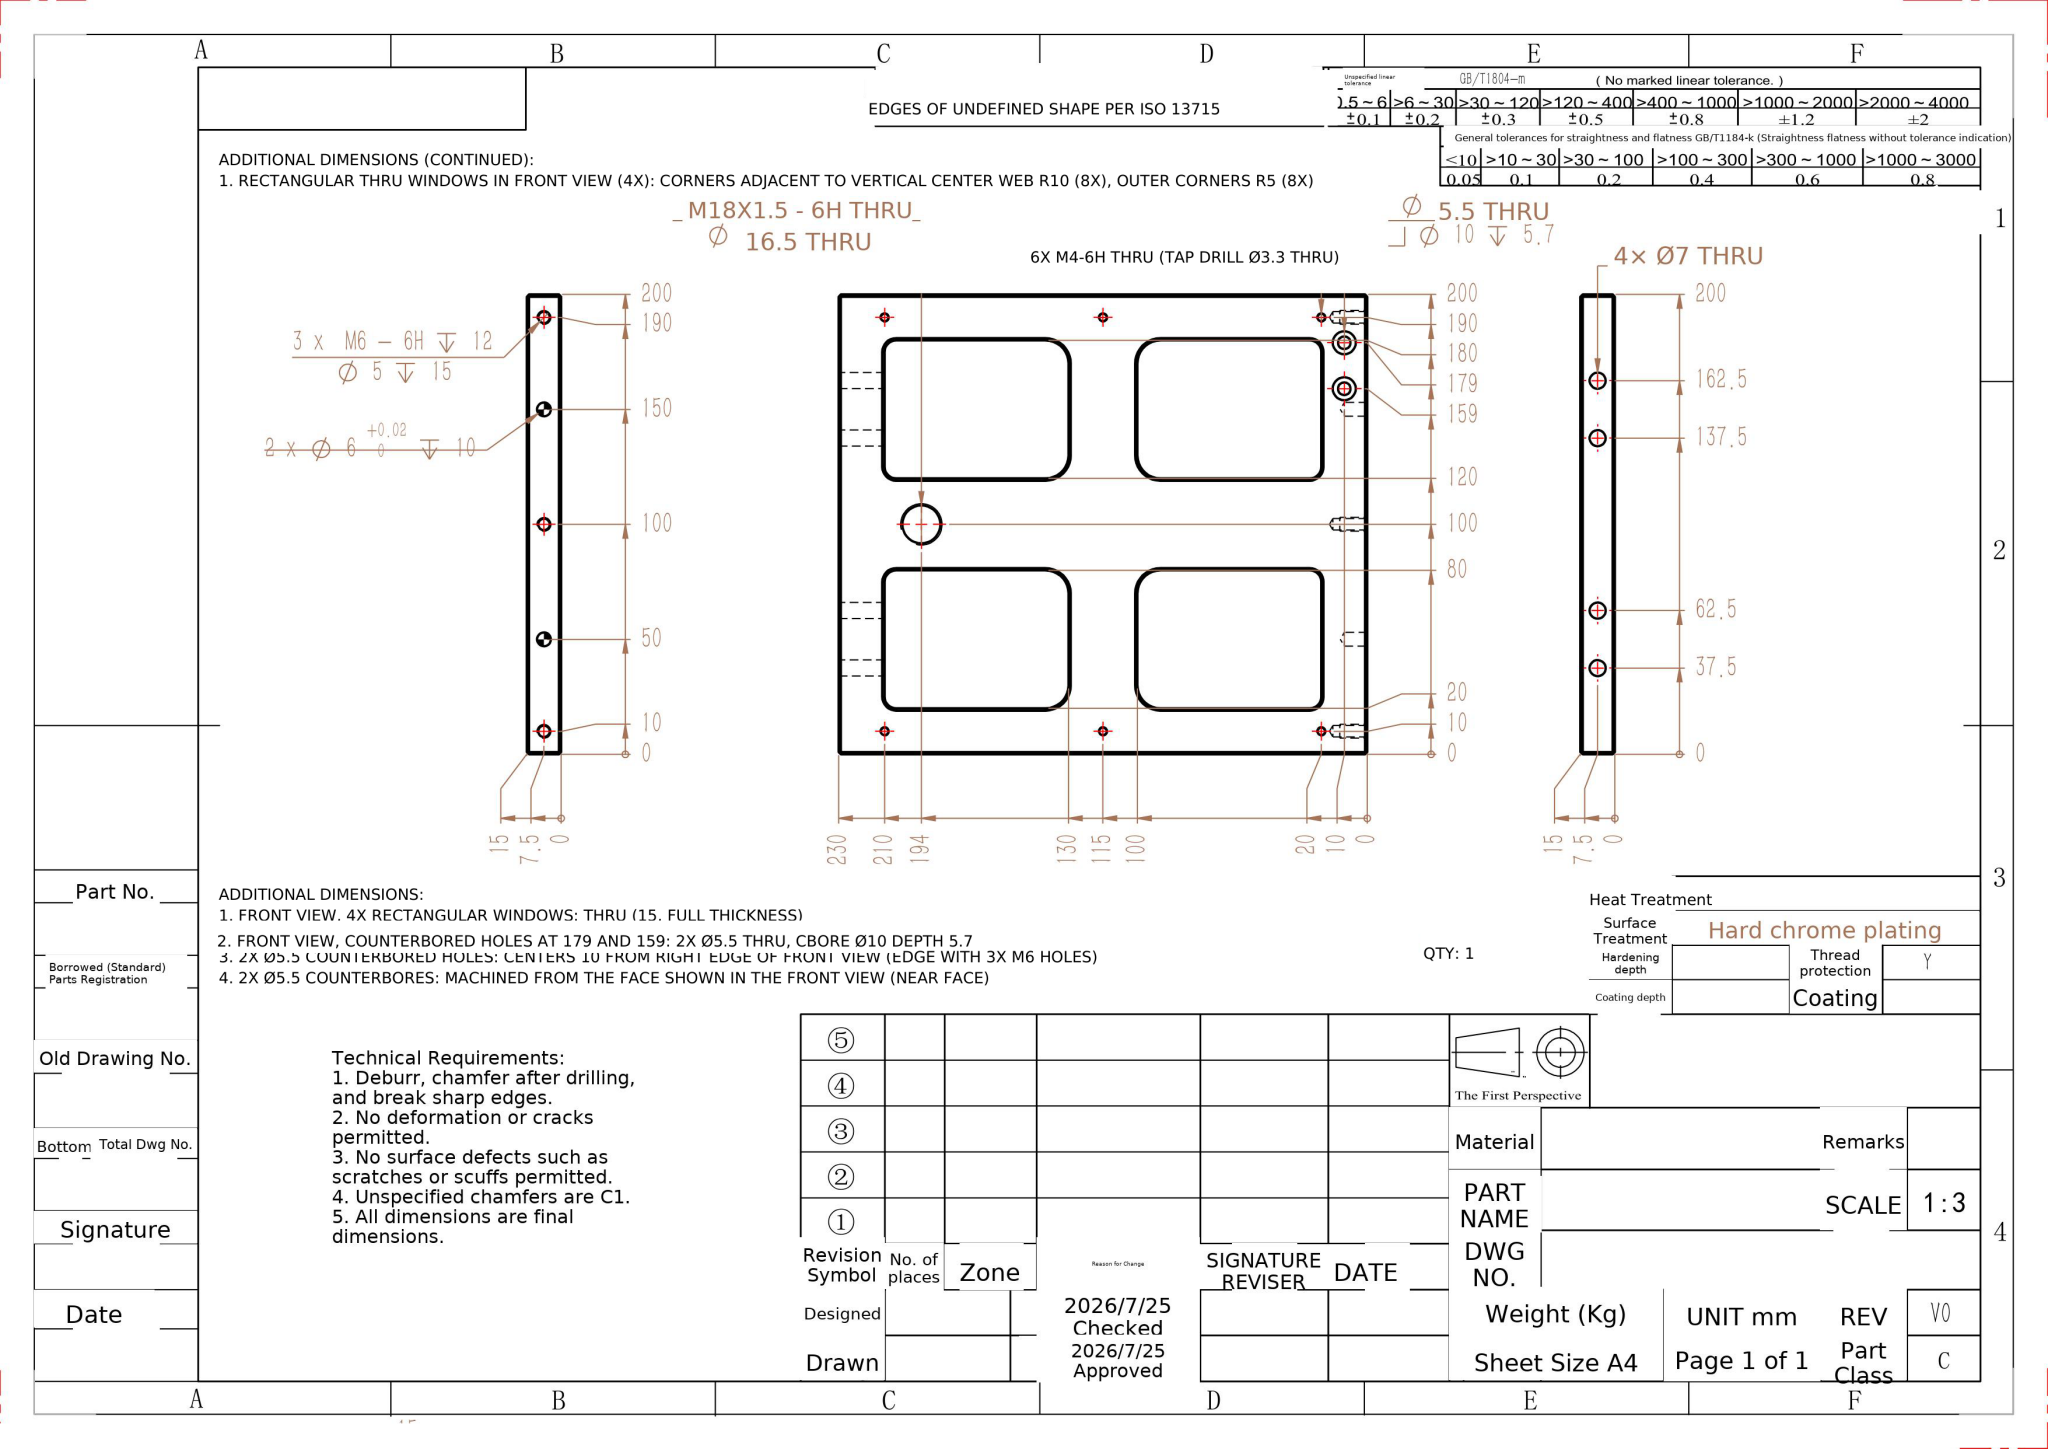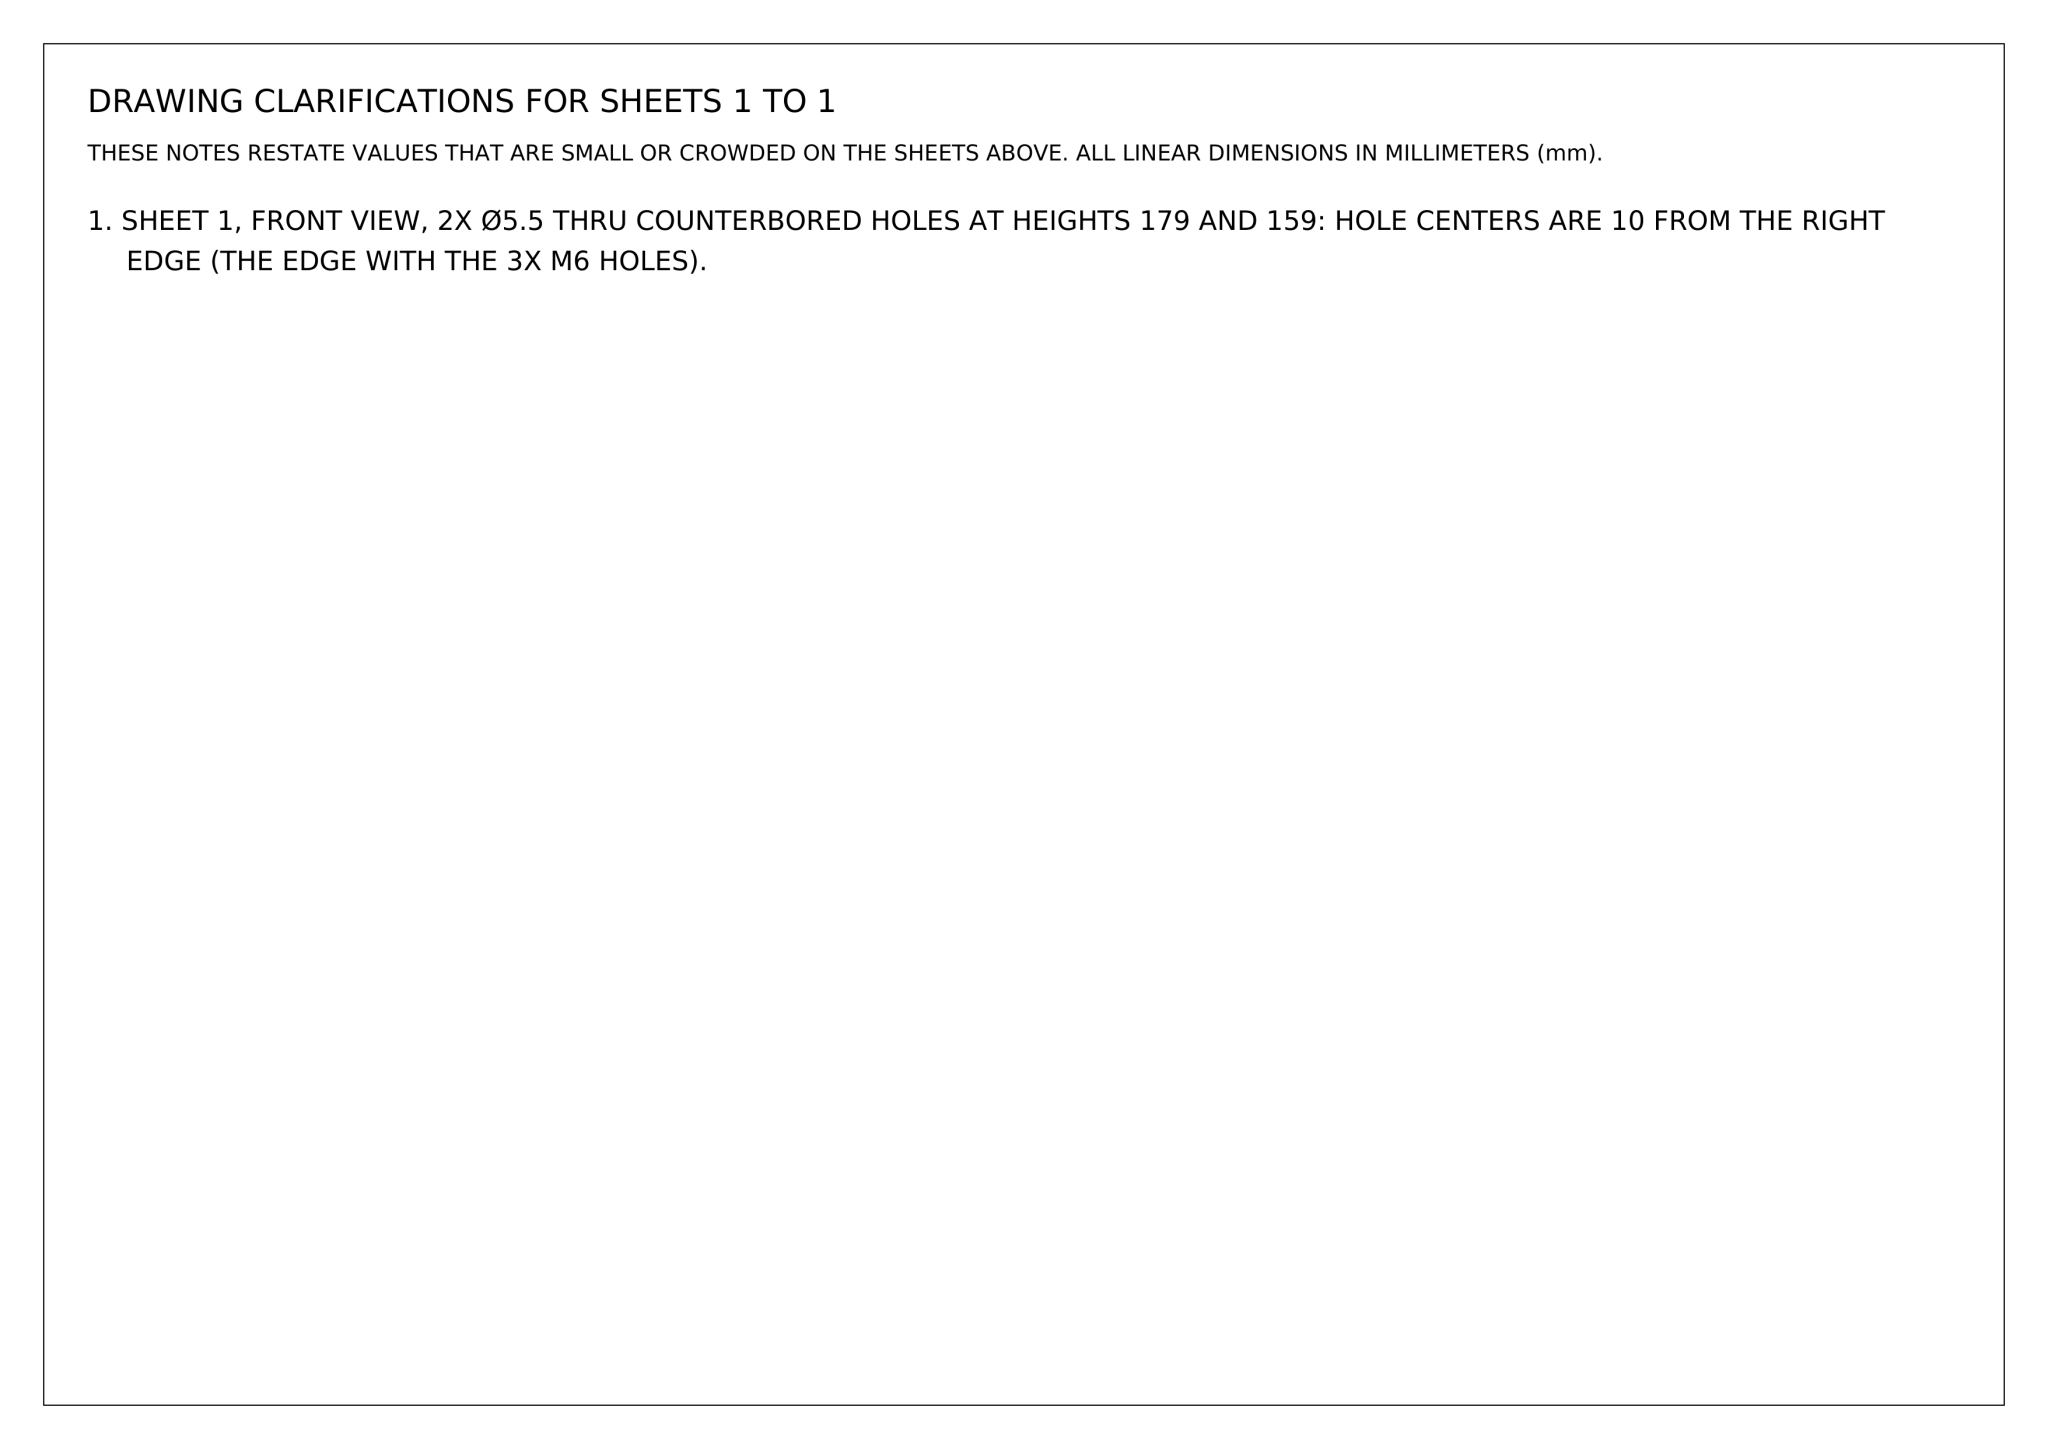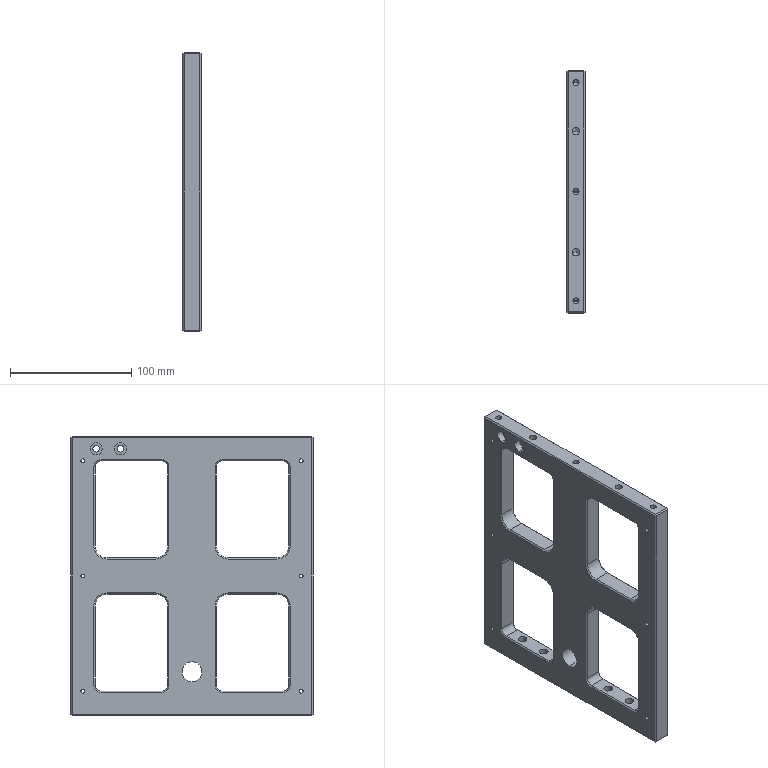Part | NX | mm | 1 solid | 174 faces | box 15 x 200 x 230 mm | volume 393352 mm3 | plane 76 | cylinder 56 | cone 42 | commonest cylinder face diameters 10 x12 3.3 x12 7 x8 20 x8 5 x6 5.5 x4 6 x4 16.5 x2